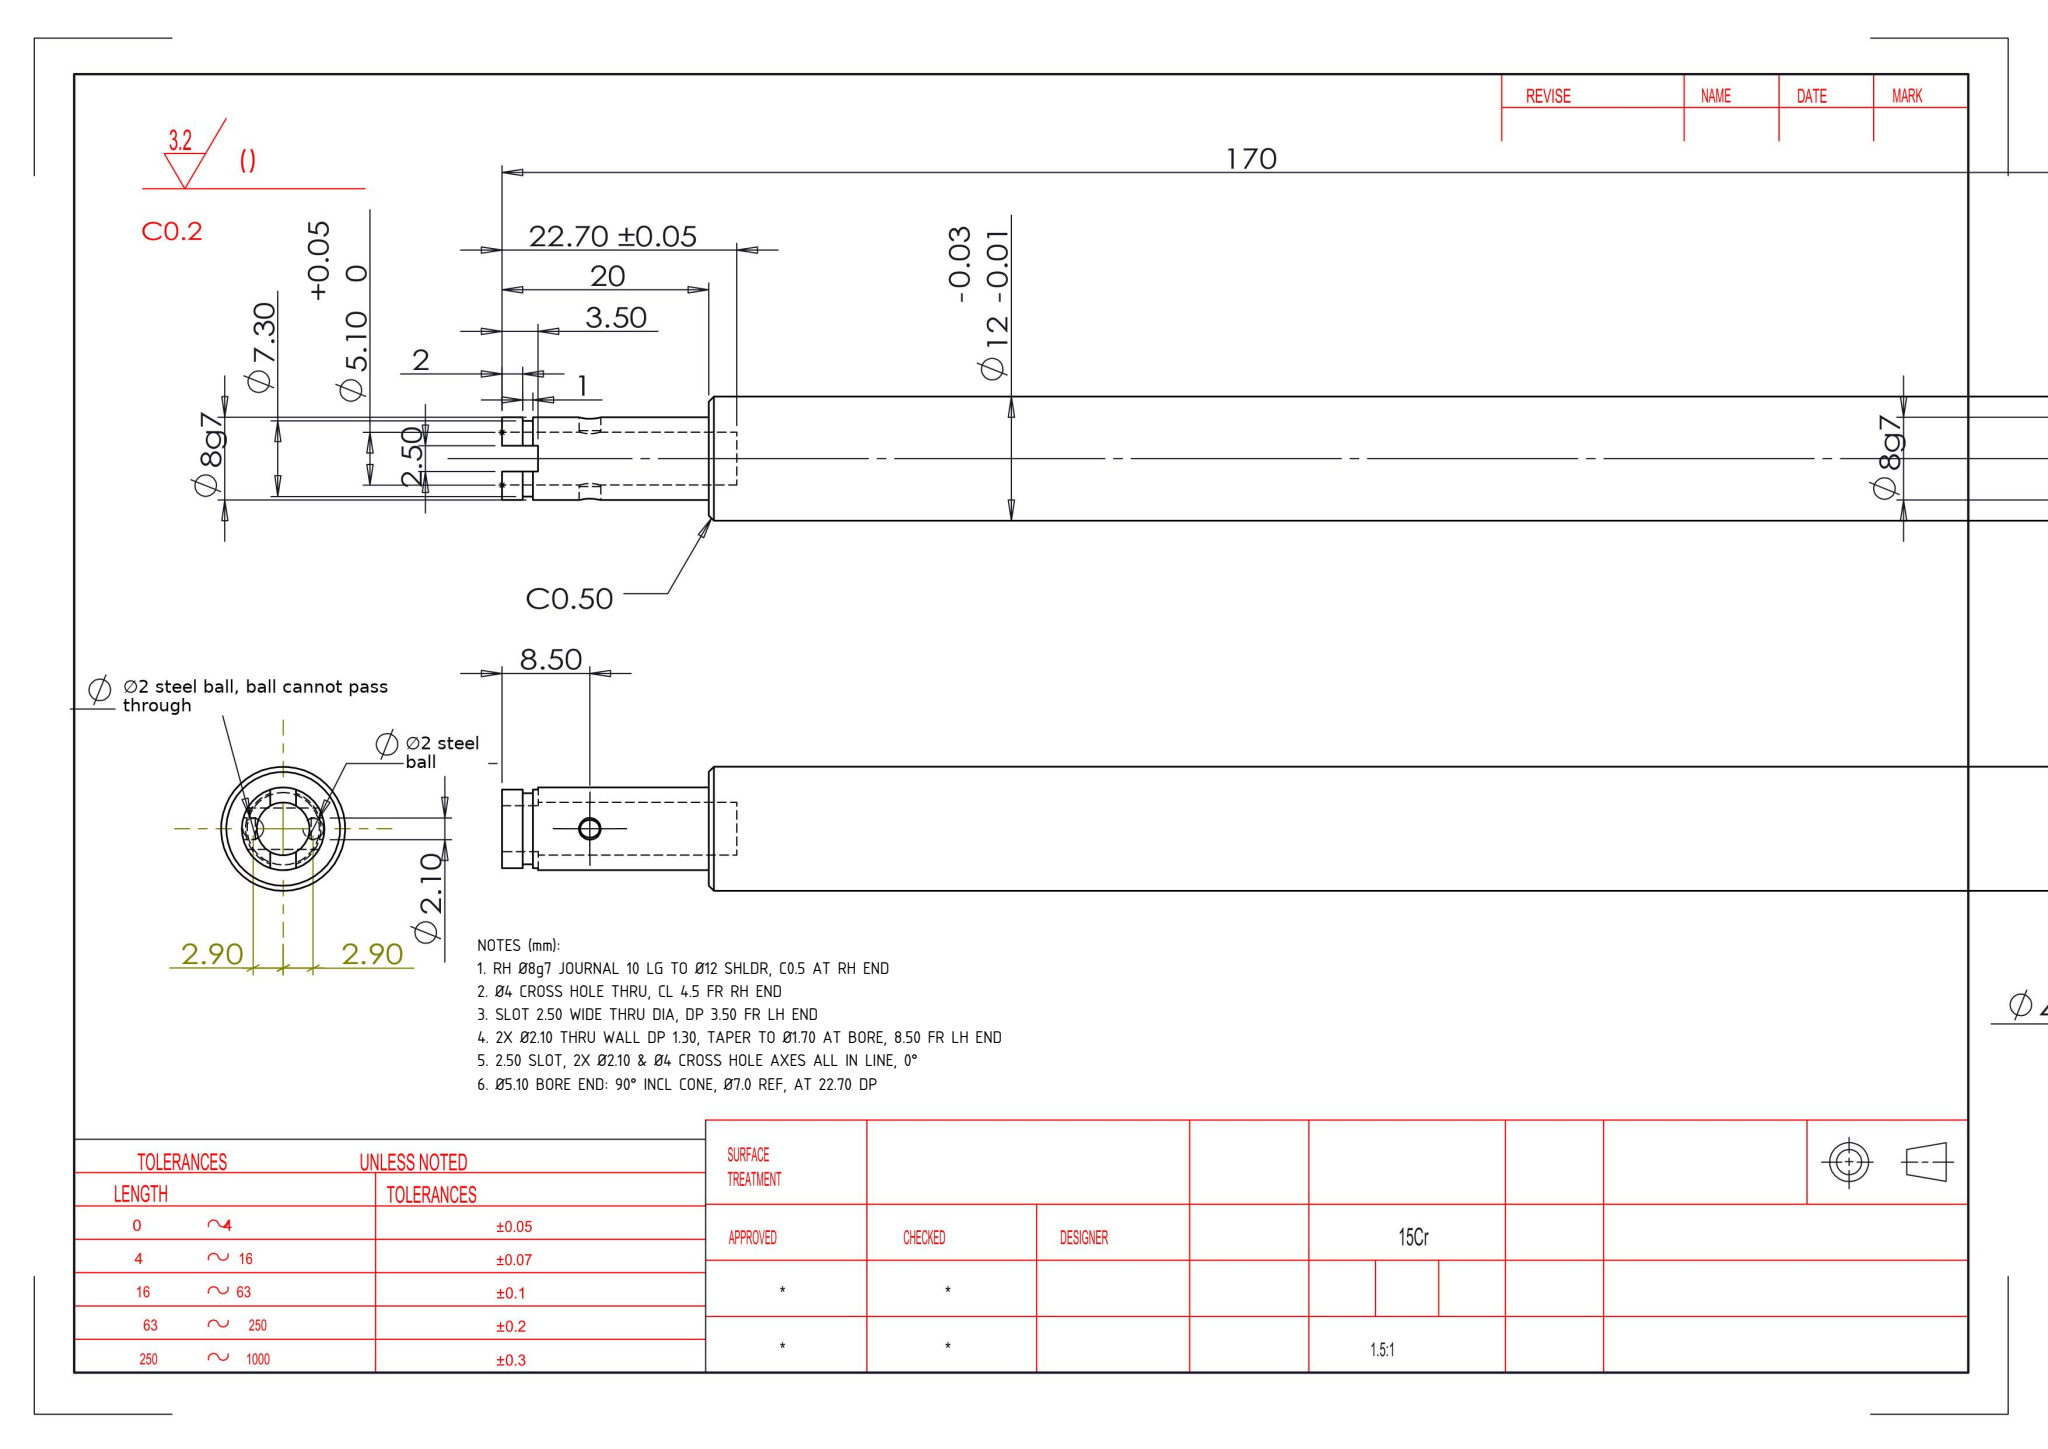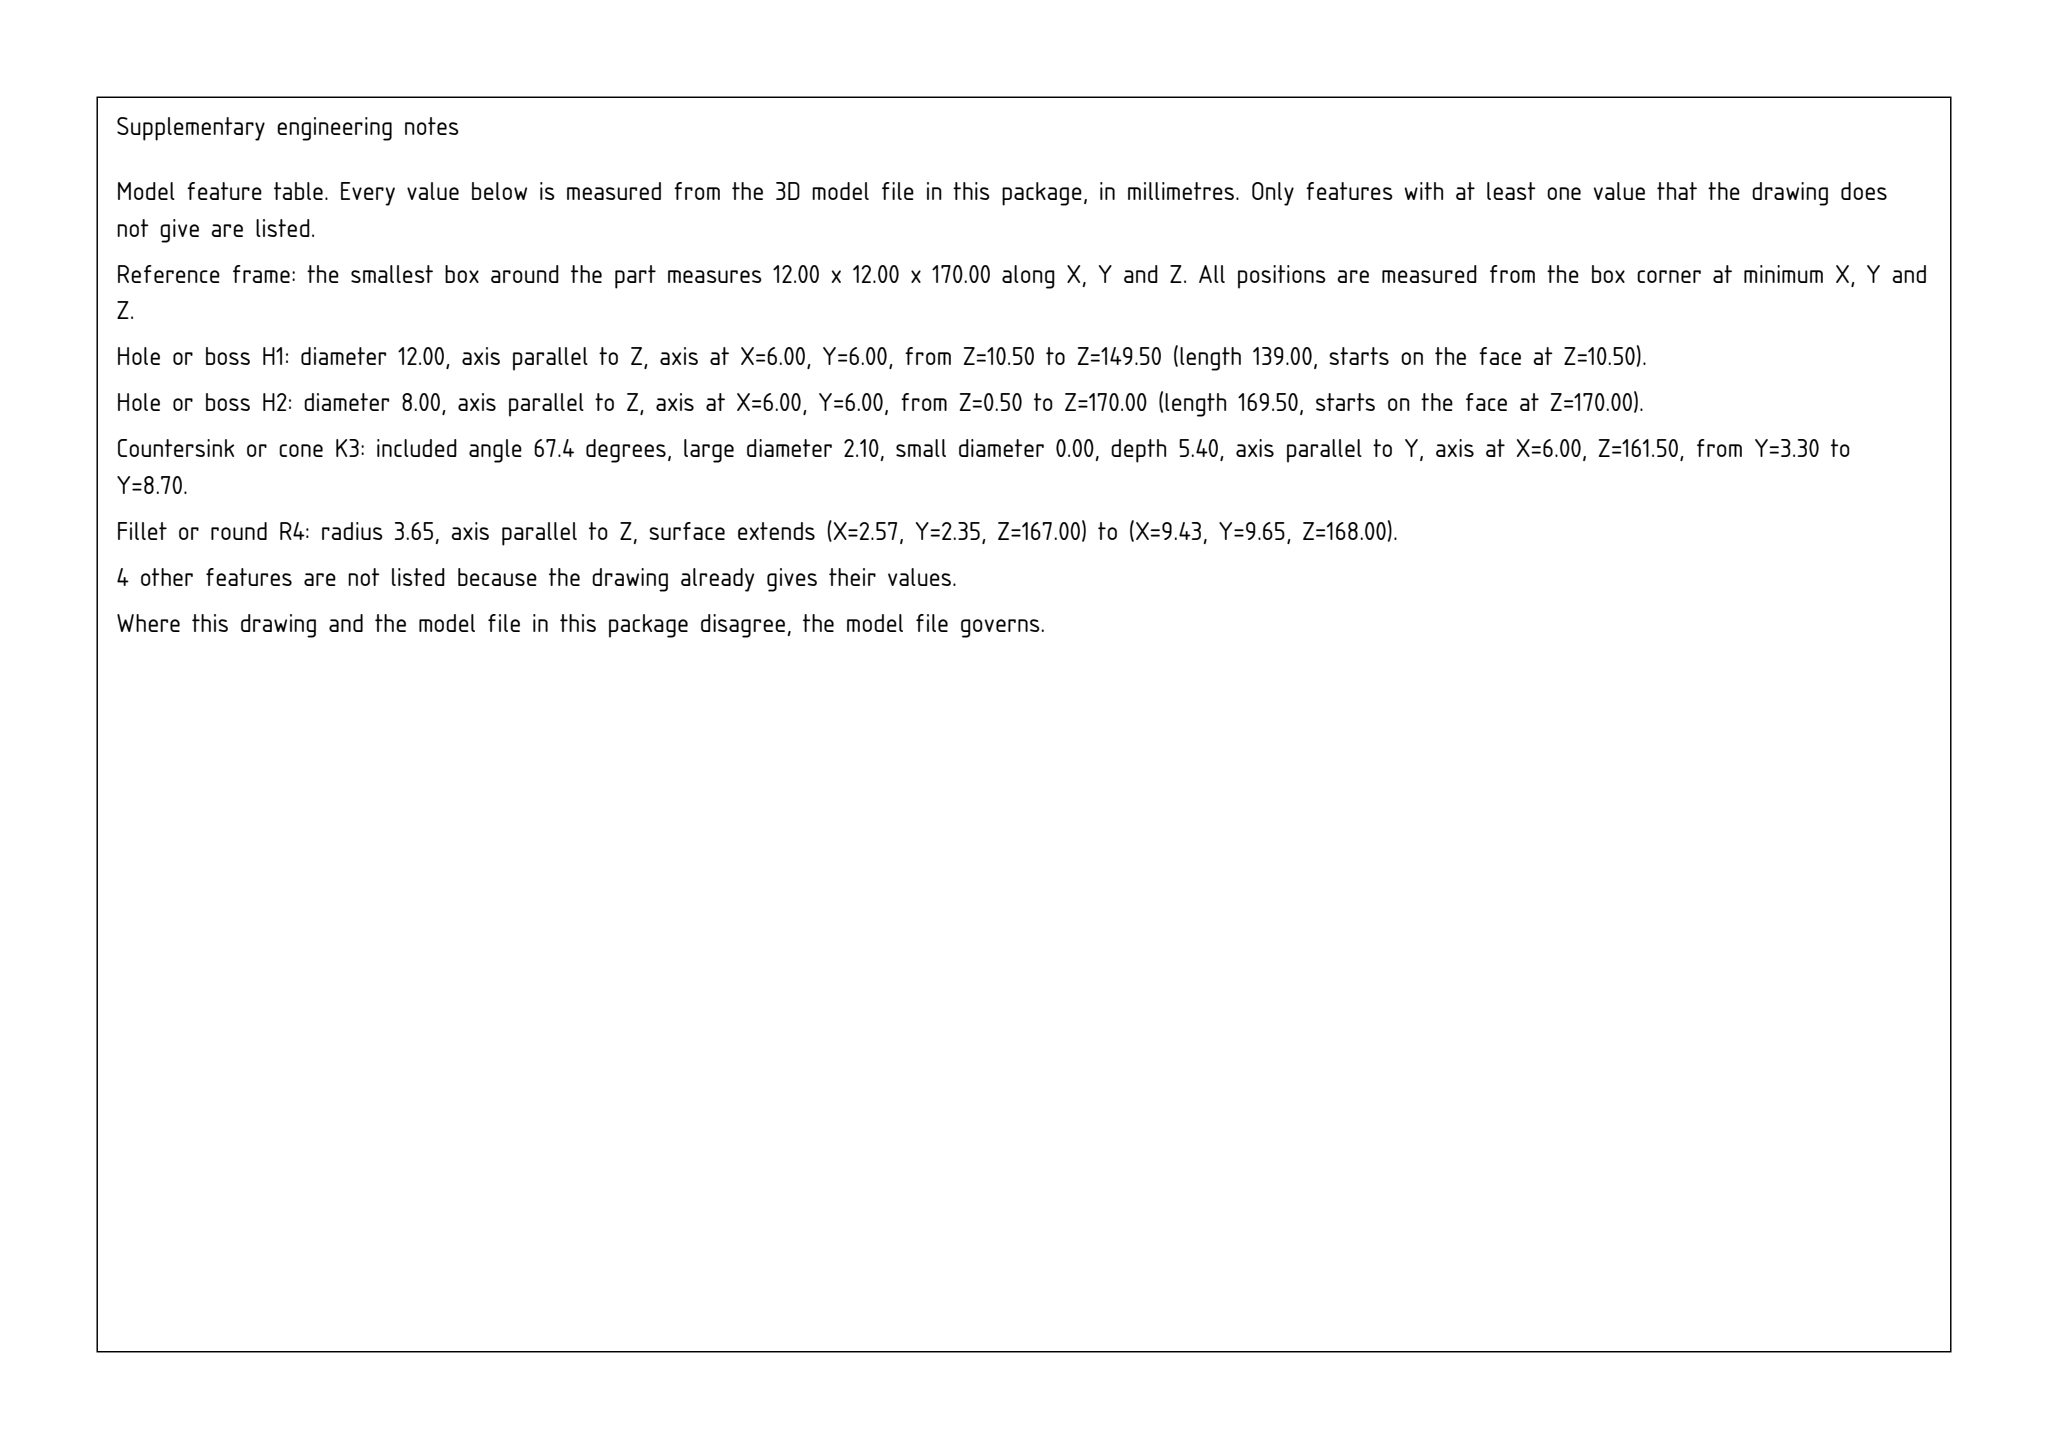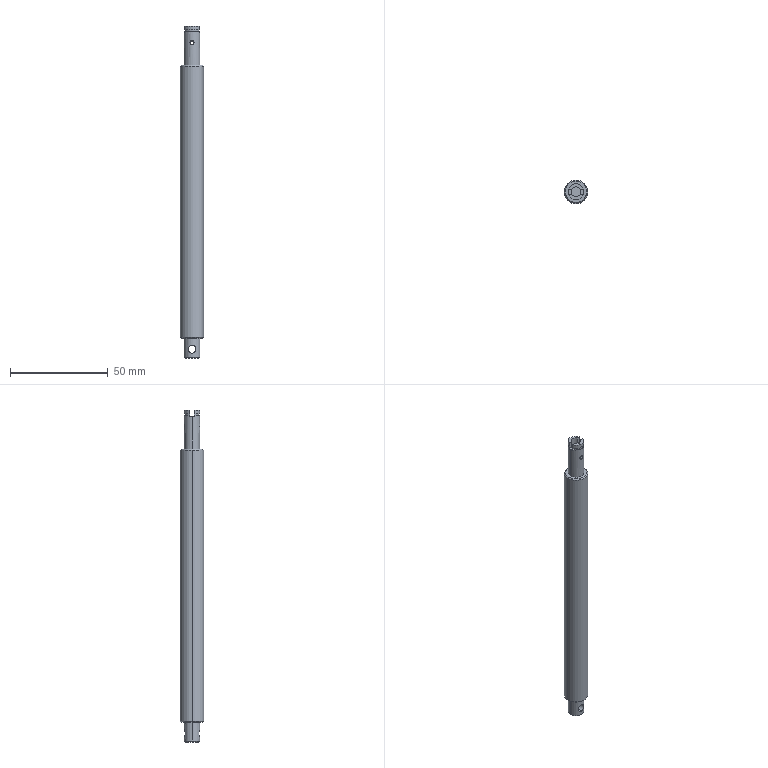Part | SolidWorks | mm | 1 solid | 44 faces | box 12 x 12 x 170 mm | volume 16726 mm3 | cylinder 18 | plane 16 | cone 10 | commonest cylinder face diameters 8 x6 2.1 x4 4 x2 12 x2 5.1 x2 7.3 x2
Drawing notes:
RH Ø8g7 JOURNAL 10 LG TO Ø12 SHLDR, C0.5 AT RH END | from the solid: Ø8 z-cyl L=9.5 from z=0.5-10 + 90° cone ref Ø7 (C0.5) at z=0; Ø12 starts z=10
Ø4 CROSS HOLE THRU, CL 4.5 FR RH END | from the solid: Ø4 y-axis cyl L=8.0 (thru Ø8) at z=4.5 from RH end z=0
SLOT 2.50 WIDE THRU DIA, DP 3.50 FR LH END | from the solid: y-planes at 4.75 & 7.25 (2.50 wide, ctr y=6); slot btm plane z=166.5 = 3.50 fr LH end z=170
2X Ø2.10 THRU WALL DP 1.30, TAPER TO Ø1.70 AT BORE, 8.50 FR LH END | from the solid: Ø2.1 y-axis cyls L=1.3 at z=161.5 (170-161.5=8.5); 67.4° cones ref Ø2.1 to Ø1.7 at bore
2.50 SLOT, 2X Ø2.10 & Ø4 CROSS HOLE AXES ALL IN LINE, 0° | from the solid: Slot faces normal Y at y=4.75/7.25 (ctr 6.0); Ø2.10 holes axis Y at x=6.0, z=161.5; Ø4 hole axis Y at x=6.0, z=4.5 - all coplanar, no angular offset
Ø5.10 BORE END: 90° INCL CONE, Ø7.0 REF, AT 22.70 DP | from the solid: cones[90.0, ref_dia 7.0] at bottom of Ø5.10 bore (bore z=147.3 to 170.0, 22.7 deep)
build123d program:
from build123d import *

# Parameters (mm, degrees)
SKETCH3_W           = 13.415
SKETCH3_H           = 2.5
EXTRUDE3_DEPTH      = 3.5
EXTRUDE4_DEPTH      = 168.727
EXTRUDE4_DEPTH_BACK = 168.727
SKETCH5_R           = 2
CHAMFER1_SIZE       = 0.5
SKETCH6_R           = 11.229
SKETCH6_R_2         = 6
CUT_EXTRUDE1_DEPTH  = 10
CHAMFER2_SIZE       = 0.5


with BuildPart() as part:
    # Sketch1 → Revolve1 (revolve)
    with BuildSketch(Plane(origin=(0, 0, 0), x_dir=(1, 0, 0), z_dir=(0, 1, 0)), mode=Mode.PRIVATE) as revolve1_sk:
        Polygon((-30.056, 162.171), (-30.056, 152.171), (-26.056, 152.171), (-26.056, 150.171), (-28.056, 150.171), (-28.056, 12.171), (-30.056, 12.171), (-30.056, -4.829), (-30.406, -4.829), (-30.406, -5.829), (-30.056, -5.829), (-30.056, -7.829), (-31.506, -7.829), (-31.506, 14.871), (-34.056, 14.871), (-34.056, 162.171), align=None)
    revolve(revolve1_sk.sketch.rotate(Axis((-34.056, 0, -29.69), (0, 0, 1)), 180), axis=Axis((-34.056, 0, -29.69), (0, 0, 1)))

    # Sketch3 → Extrude3 (cut)
    with BuildSketch(Plane.XY.offset(7.829)):
        with Locations((-34.201, 0)):
            Rectangle(SKETCH3_W, SKETCH3_H)
    extrude(amount=-EXTRUDE3_DEPTH, mode=Mode.SUBTRACT)

    # Sketch4 → Cut-Revolve4 (revolve, cut)
    with BuildSketch(Plane(origin=(-34.056, 0, 0), x_dir=(0, 0, -1), z_dir=(1, 0, 0)), mode=Mode.PRIVATE) as cut_revolve4_sk:
        Polygon((1.721, -4.489), (1.721, -2.7), (1.521, -2.4), (0.6714, -2.4), (0.6714, -4.489), align=None)
        Polygon((1.721, 4.564), (0.6714, 4.564), (0.6714, 2.4), (1.521, 2.4), (1.721, 2.7), align=None)
    revolve(cut_revolve4_sk.sketch.rotate(Axis((-34.056, 6.692, -0.6714), (0, -1, 0)), 270), axis=Axis((-34.056, 6.692, -0.6714), (0, -1, 0)), mode=Mode.SUBTRACT)

    # Sketch5 → Extrude4 (cut, two sides: drawn at the far end of the back side and taken through both)
    with BuildSketch(Plane(origin=(0, 0, 0), x_dir=(1, 0, 0), z_dir=(0, 1, 0)).offset(-EXTRUDE4_DEPTH_BACK)):
        with Locations(Location((-34.056, 157.671, 0), (0, 0, 270))):
            Circle(SKETCH5_R)
    extrude(amount=EXTRUDE4_DEPTH + EXTRUDE4_DEPTH_BACK, mode=Mode.SUBTRACT)

    # Chamfer1
    chamfer1_edges = [part.edges().sort_by_distance(p)[0] for p in [
        (-30.056, 0, -162.171),
        (-28.056, 0, -12.171),
    ]]
    chamfer(chamfer1_edges, length=CHAMFER1_SIZE)

    # Sketch6 → Cut-Extrude1 (cut)
    with BuildSketch(Plane.XY.offset(-150.171)):
        with Locations((-34.056, 0)):
            Circle(SKETCH6_R)
        with Locations(Location((-34.056, 0, 0), (0, 0, 180))):
            Circle(SKETCH6_R_2, mode=Mode.SUBTRACT)
    extrude(amount=-CUT_EXTRUDE1_DEPTH, mode=Mode.SUBTRACT)

    # Chamfer2
    chamfer2_edges = [part.edges().sort_by_distance(p)[0] for p in [
        (-28.056, 0, -152.171),
    ]]
    chamfer(chamfer2_edges, length=CHAMFER2_SIZE)


solid = part.part